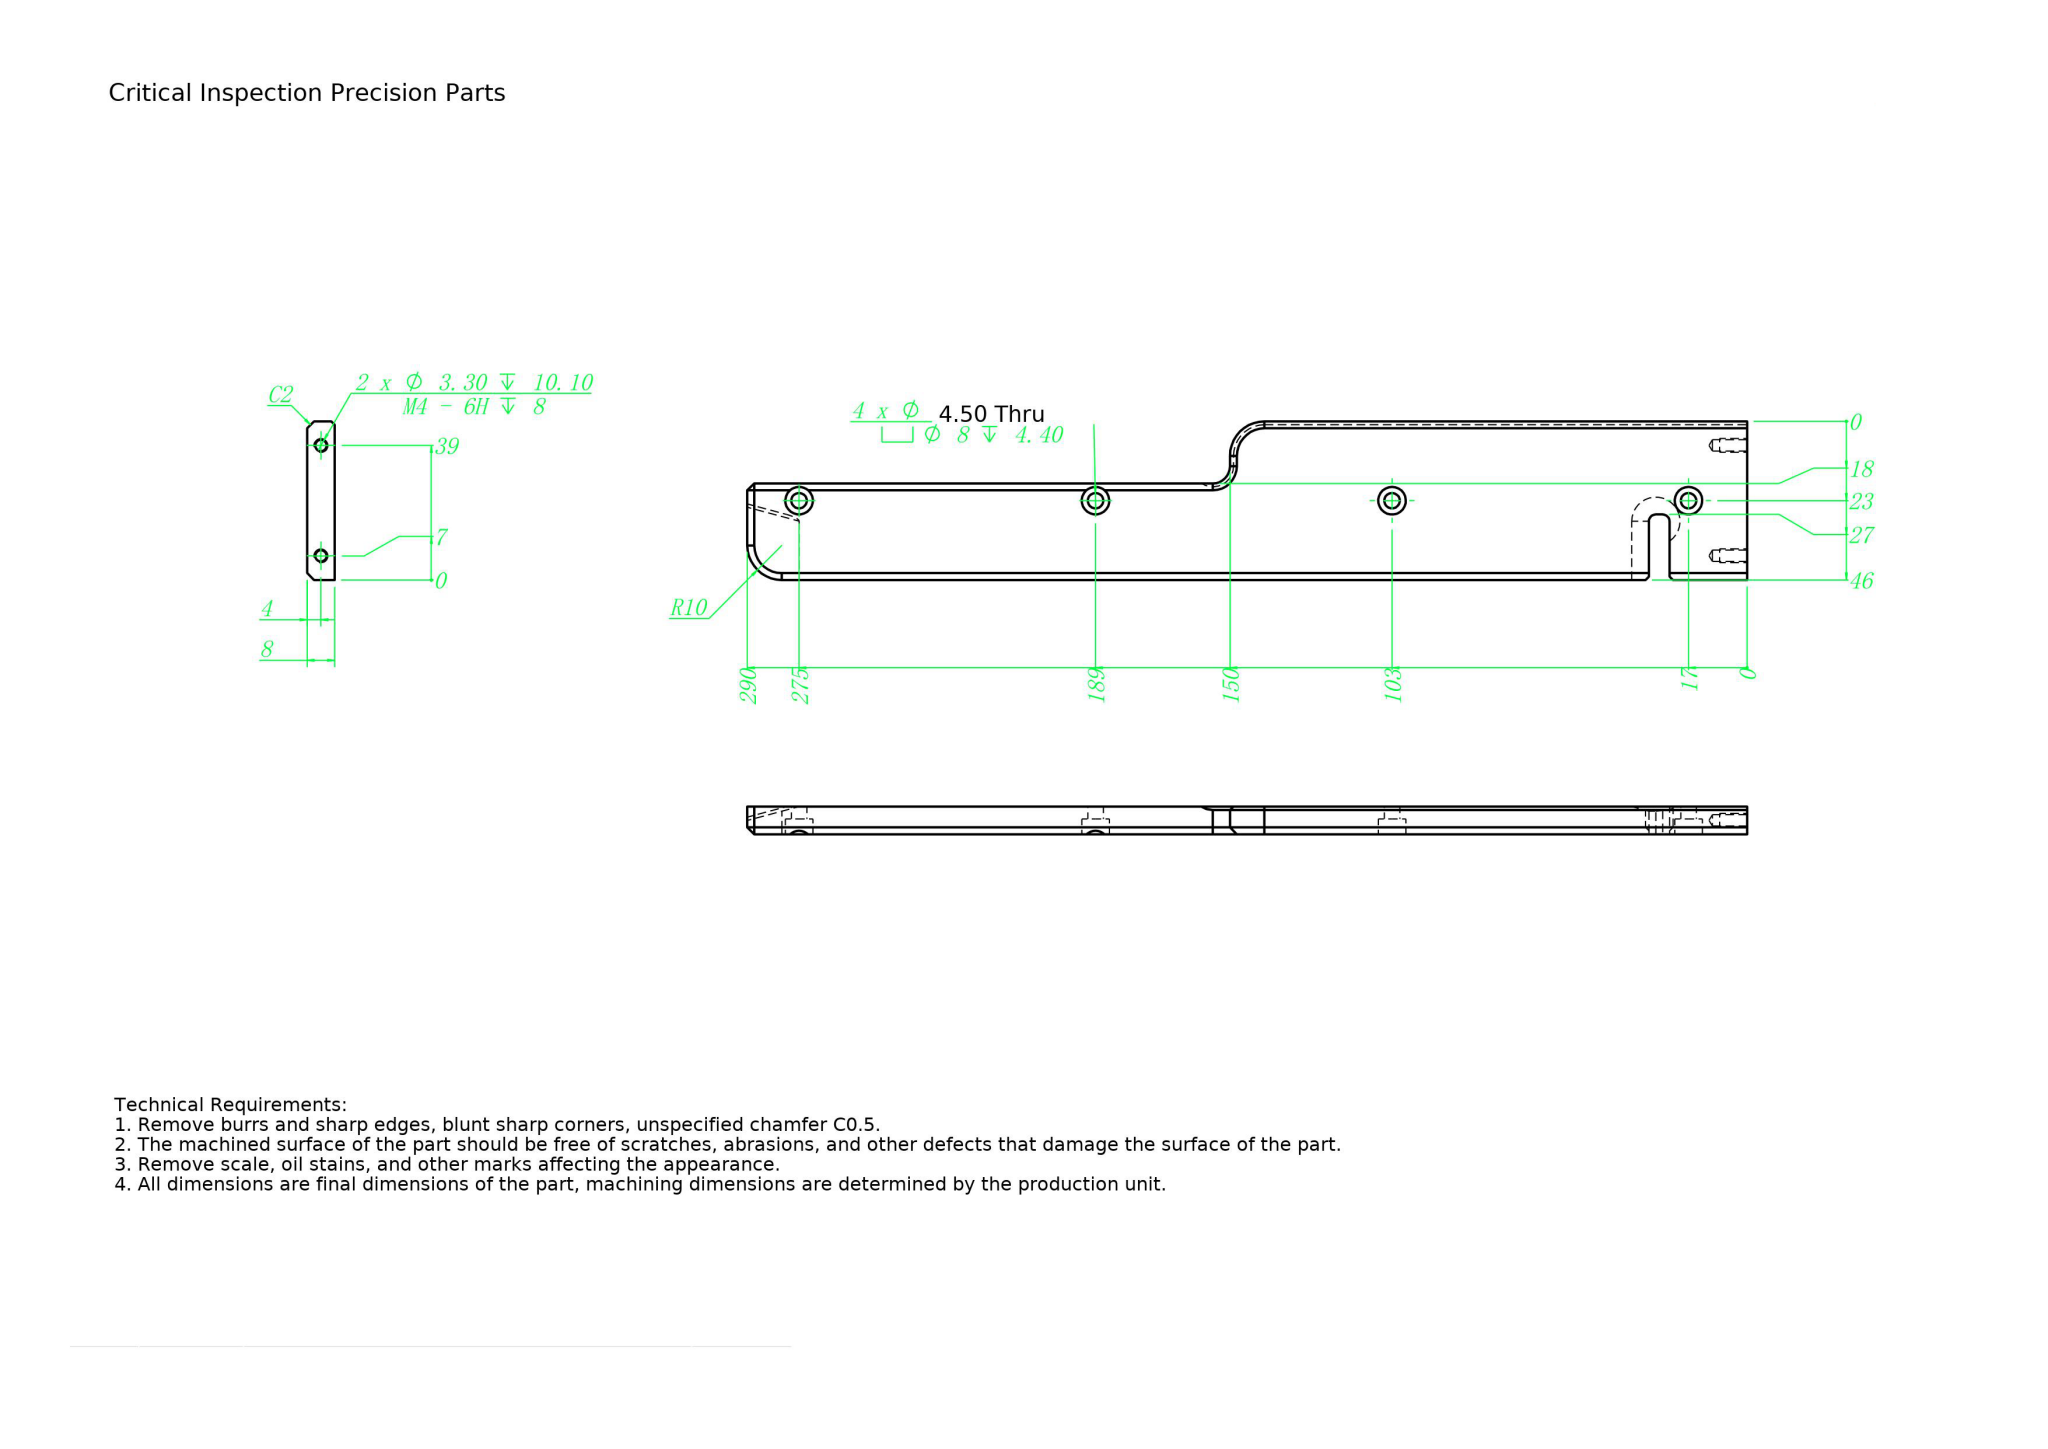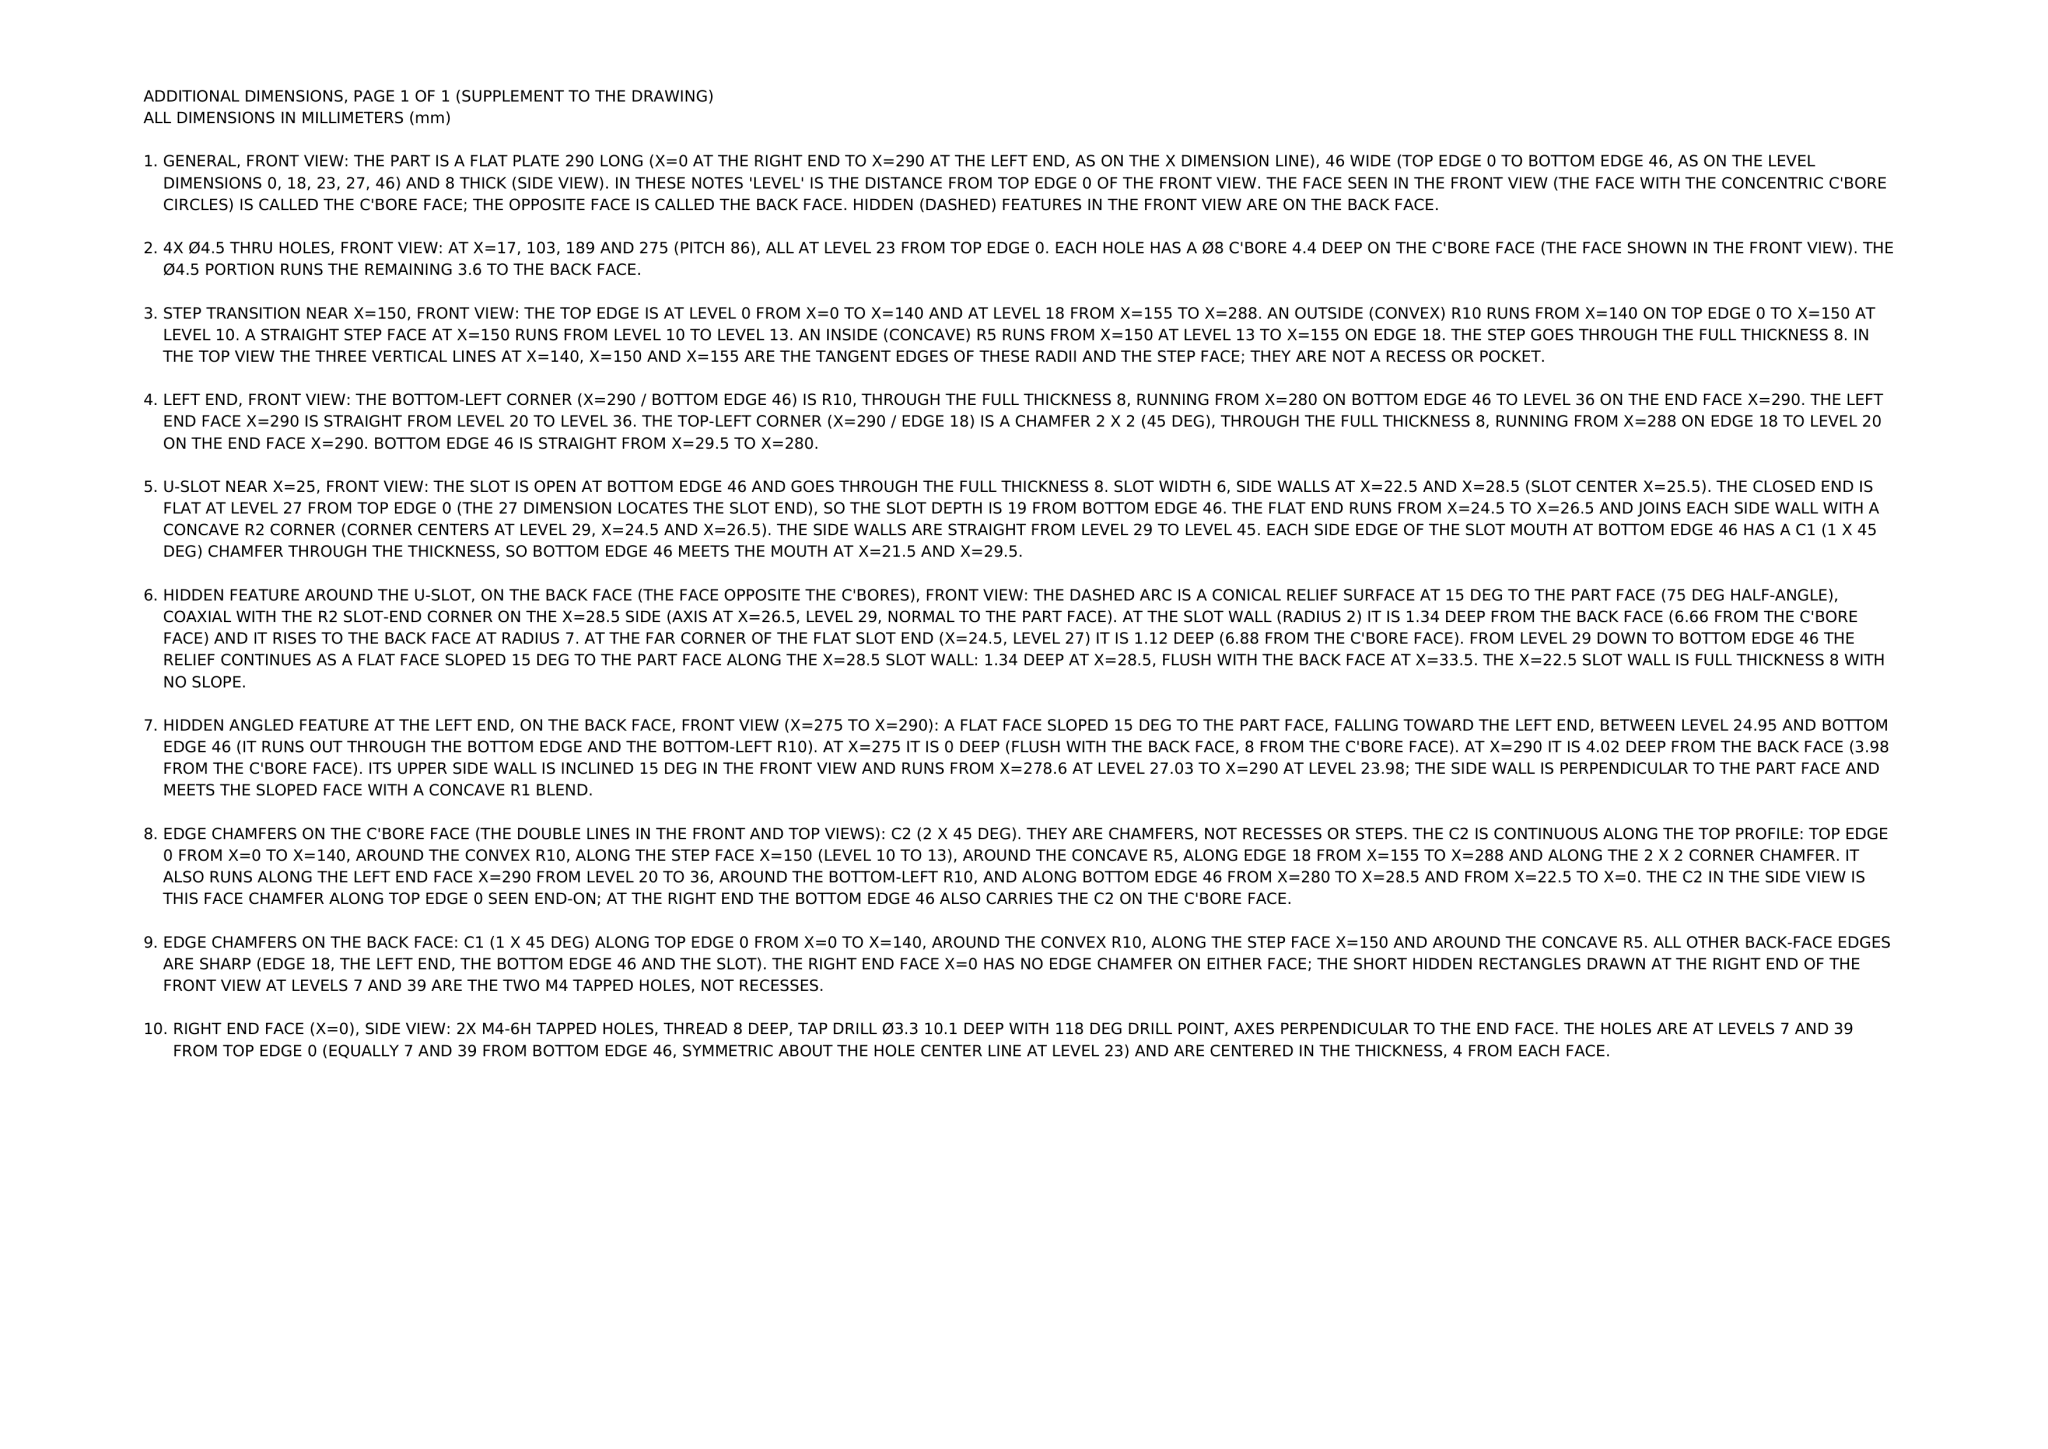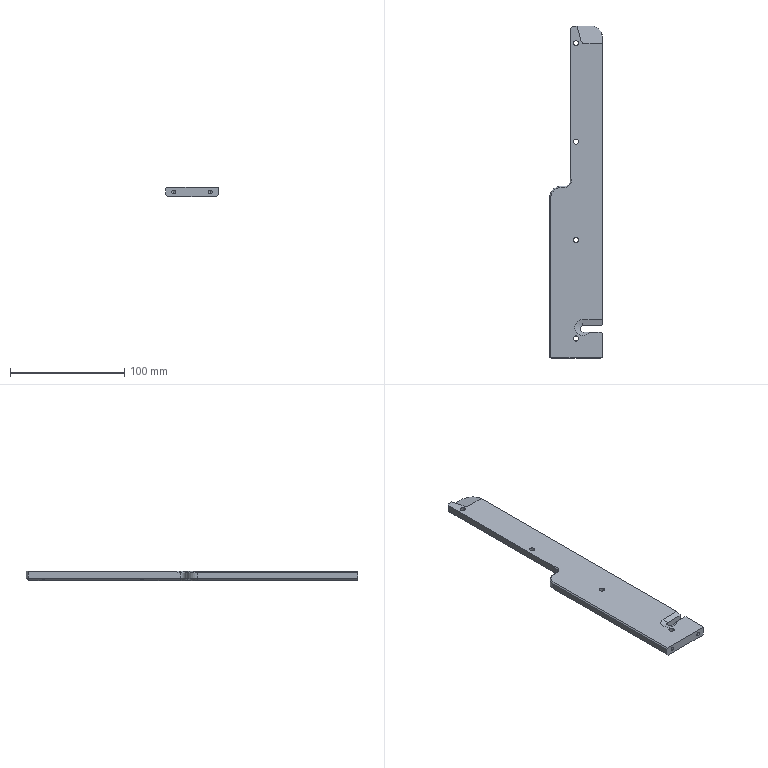Part | NX | mm | 1 solid | 68 faces | box 46 x 290 x 8 mm | volume 82113 mm3 | plane 31 | cylinder 26 | cone 11 | commonest cylinder face diameters 8 x8 4.5 x8 3.3 x4 20 x2 4 x2 10 x1 2 x1